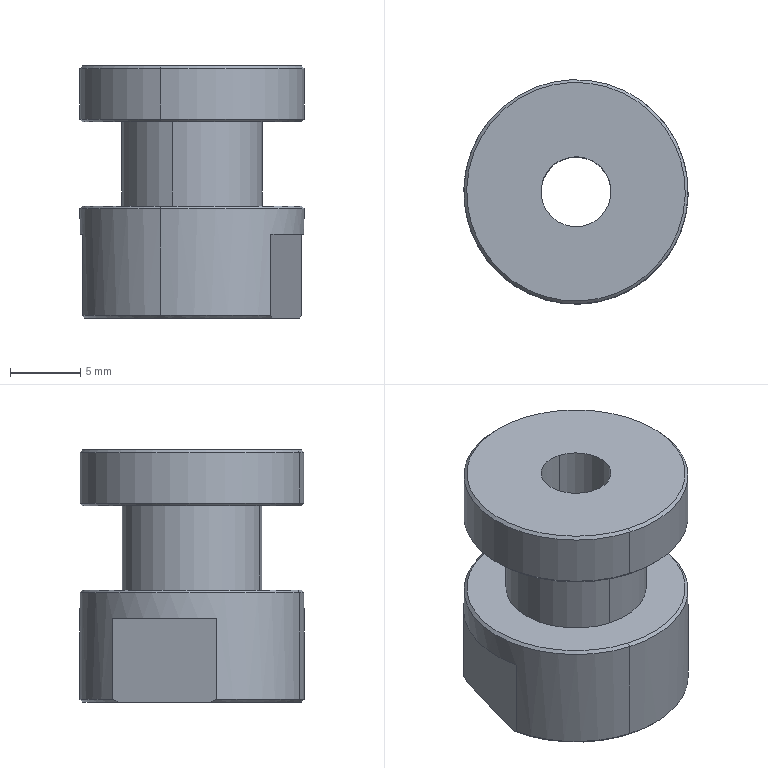Component | SolidWorks | 002MaterialPickingModuleA-1_004SidePlugModule-1_J-012-1 | 1 solid | 25 faces | box 16 x 16 x 18 mm | volume 2464 mm3 | cone 9 | cylinder 8 | plane 8 | commonest cylinder face diameters 16 x4 5 x2 10 x2 | material 45
build123d program:
from build123d import *

# Parameters (mm, degrees)
M6_TAPPED_HOLE1_D  = 5
CUT_EXTRUDE1_DEPTH = 6
CHAMFER1_SIZE      = 0.2


with BuildPart() as part:
    # Sketch2 → Revolve1 (revolve)
    with BuildSketch(Plane.XY, mode=Mode.PRIVATE) as revolve1_sk:
        Polygon((0, 0), (0, 8), (4, 8), (4, 5), (10, 5), (10, 8), (18, 8), (18, 0), align=None)
    revolve(revolve1_sk.sketch.rotate(Axis((0, 0, 0), (1, 0, 0)), 90), axis=Axis((0, 0, 0), (1, 0, 0)))

    # M6 Tapped Hole1 (through all)
    with Locations(Plane(origin=(18, 0, 0), x_dir=(0, 0, -1), z_dir=(1, 0, 0))):
        with Locations((0, 0)):
            Hole(M6_TAPPED_HOLE1_D / 2)

    # Sketch5 → Cut-Extrude1 (cut)
    with BuildSketch(Plane(origin=(18, 0, 0), x_dir=(0, 0, -1), z_dir=(1, 0, 0))):
        with BuildLine():
            Line((3.873, -7), (-3.873, -7))
            ThreePointArc((-3.873, -7), (0, -8), (3.873, -7))
        make_face()
        with BuildLine():
            Line((3.873, 7), (-3.873, 7))
            ThreePointArc((-3.873, 7), (0, 8), (3.873, 7))
        make_face()
    extrude(amount=-CUT_EXTRUDE1_DEPTH, mode=Mode.SUBTRACT)

    # Chamfer1
    chamfer1_edges = [part.edges().sort_by_distance(p)[0] for p in [
        (18, 0, -8),
        (18, -4.063, 6.891),
        (10, 0, -8),
        (4, 0, -8),
        (0, 0, -8),
    ]]
    chamfer(chamfer1_edges, length=CHAMFER1_SIZE)


solid = part.part

# Placed as in the assembly
solid = solid.moved(Location((220.325, 319.019, 480.731), (-90, 16.272, 90)))
STEP:
#1=COLOUR_RGB('',0.7922,0.8196,0.9333);
#2=FILL_AREA_STYLE_COLOUR('',#1);
#3=FILL_AREA_STYLE('',(#2));
#4=SURFACE_STYLE_FILL_AREA(#3);
#5=SURFACE_SIDE_STYLE('',(#4));
#6=SURFACE_STYLE_USAGE(.BOTH.,#5);
#7=PRESENTATION_STYLE_ASSIGNMENT((#6));
#8=CARTESIAN_POINT('',(8.76,12.855,18.218));
#9=VERTEX_POINT('',#8);
#10=CARTESIAN_POINT('',(8.977,12.613,18.218));
#11=VERTEX_POINT('',#10);
#12=CARTESIAN_POINT('',(8.674,12.56,18.218));
#13=DIRECTION('',(0.,0.,-1.));
#14=DIRECTION('',(0.2802,0.9599,0.));
#15=AXIS2_PLACEMENT_3D('',#12,#13,#14);
#16=CIRCLE('',#15,0.3071);
#17=EDGE_CURVE('',#9,#11,#16,.T.);
#18=ORIENTED_EDGE('',*,*,#17,.F.);
#19=CARTESIAN_POINT('',(8.762,12.862,18.226));
#20=VERTEX_POINT('',#19);
#21=CARTESIAN_POINT('',(8.762,12.862,18.226));
#22=DIRECTION('',(0.1981,0.6788,0.7071));
#23=VECTOR('',#22,39.37);
#24=LINE('',#21,#23);
#25=EDGE_CURVE('',#9,#20,#24,.T.);
#26=ORIENTED_EDGE('',*,*,#25,.T.);
#27=CARTESIAN_POINT('',(8.981,12.629,18.226));
#28=VERTEX_POINT('',#27);
#29=CARTESIAN_POINT('',(8.674,12.56,18.226));
#30=DIRECTION('',(0.,0.,1.));
#31=DIRECTION('',(0.2802,0.9599,0.));
#32=AXIS2_PLACEMENT_3D('',#29,#30,#31);
#33=CIRCLE('',#32,0.315);
#34=EDGE_CURVE('',#28,#20,#33,.T.);
#35=ORIENTED_EDGE('',*,*,#34,.F.);
#36=CARTESIAN_POINT('',(8.977,12.613,18.218));
#37=CARTESIAN_POINT('',(8.978,12.618,18.22));
#38=CARTESIAN_POINT('',(8.98,12.624,18.223));
#39=CARTESIAN_POINT('',(8.981,12.629,18.226));
#40=B_SPLINE_CURVE_WITH_KNOTS('',3,(#36,#37,#38,#39),.UNSPECIFIED.,.F.,.F.,(4,4),(0.,0.0004761),.UNSPECIFIED.);
#41=EDGE_CURVE('',#11,#28,#40,.T.);
#42=ORIENTED_EDGE('',*,*,#41,.F.);
#43=EDGE_LOOP('',(#18,#26,#35,#42));
#44=FACE_OUTER_BOUND('',#43,.T.);
#45=CARTESIAN_POINT('',(8.674,12.56,18.226));
#46=DIRECTION('',(0.,0.,1.));
#47=DIRECTION('',(0.2802,0.9599,0.));
#48=AXIS2_PLACEMENT_3D('',#45,#46,#47);
#49=CONICAL_SURFACE('',#48,0.315,0.7854);
#50=ADVANCED_FACE('',(#44),#49,.T.);
#51=CARTESIAN_POINT('',(8.76,12.855,18.533));
#52=VERTEX_POINT('',#51);
#53=CARTESIAN_POINT('',(8.588,12.265,18.533));
#54=VERTEX_POINT('',#53);
#55=CARTESIAN_POINT('',(8.674,12.56,18.533));
#56=DIRECTION('',(0.,0.,1.));
#57=DIRECTION('',(-0.2802,-0.9599,0.));
#58=AXIS2_PLACEMENT_3D('',#55,#56,#57);
#59=CIRCLE('',#58,0.3071);
#60=EDGE_CURVE('',#52,#54,#59,.T.);
#61=ORIENTED_EDGE('',*,*,#60,.F.);
#62=CARTESIAN_POINT('',(8.762,12.862,18.525));
#63=VERTEX_POINT('',#62);
#64=CARTESIAN_POINT('',(8.76,12.855,18.533));
#65=DIRECTION('',(0.1981,0.6788,-0.7071));
#66=VECTOR('',#65,39.37);
#67=LINE('',#64,#66);
#68=EDGE_CURVE('',#52,#63,#67,.T.);
#69=ORIENTED_EDGE('',*,*,#68,.T.);
#70=CARTESIAN_POINT('',(8.586,12.257,18.525));
#71=VERTEX_POINT('',#70);
#72=CARTESIAN_POINT('',(8.674,12.56,18.525));
#73=DIRECTION('',(0.,0.,-1.));
#74=DIRECTION('',(-0.2802,-0.9599,0.));
#75=AXIS2_PLACEMENT_3D('',#72,#73,#74);
#76=CIRCLE('',#75,0.315);
#77=EDGE_CURVE('',#71,#63,#76,.T.);
#78=ORIENTED_EDGE('',*,*,#77,.F.);
#79=CARTESIAN_POINT('',(8.588,12.265,18.533));
#80=DIRECTION('',(-0.1981,-0.6788,-0.7071));
#81=VECTOR('',#80,39.37);
#82=LINE('',#79,#81);
#83=EDGE_CURVE('',#54,#71,#82,.T.);
#84=ORIENTED_EDGE('',*,*,#83,.F.);
#85=EDGE_LOOP('',(#61,#69,#78,#84));
#86=FACE_OUTER_BOUND('',#85,.T.);
#87=CARTESIAN_POINT('',(8.674,12.56,18.533));
#88=DIRECTION('',(0.,0.,-1.));
#89=DIRECTION('',(-0.2802,-0.9599,0.));
#90=AXIS2_PLACEMENT_3D('',#87,#88,#89);
#91=CONICAL_SURFACE('',#90,0.3071,0.7854);
#92=ADVANCED_FACE('',(#86),#91,.T.);
#93=CARTESIAN_POINT('',(8.588,12.265,18.769));
#94=VERTEX_POINT('',#93);
#95=CARTESIAN_POINT('',(8.76,12.855,18.769));
#96=VERTEX_POINT('',#95);
#97=CARTESIAN_POINT('',(8.674,12.56,18.769));
#98=DIRECTION('',(0.,0.,-1.));
#99=DIRECTION('',(0.2802,0.9599,0.));
#100=AXIS2_PLACEMENT_3D('',#97,#98,#99);
#101=CIRCLE('',#100,0.3071);
#102=EDGE_CURVE('',#94,#96,#101,.T.);
#103=ORIENTED_EDGE('',*,*,#102,.F.);
#104=CARTESIAN_POINT('',(8.586,12.257,18.777));
#105=VERTEX_POINT('',#104);
#106=CARTESIAN_POINT('',(8.586,12.257,18.777));
#107=DIRECTION('',(-0.1981,-0.6788,0.7071));
#108=VECTOR('',#107,39.37);
#109=LINE('',#106,#108);
#110=EDGE_CURVE('',#94,#105,#109,.T.);
#111=ORIENTED_EDGE('',*,*,#110,.T.);
#112=CARTESIAN_POINT('',(8.762,12.862,18.777));
#113=VERTEX_POINT('',#112);
#114=CARTESIAN_POINT('',(8.674,12.56,18.777));
#115=DIRECTION('',(0.,0.,1.));
#116=DIRECTION('',(0.2802,0.9599,0.));
#117=AXIS2_PLACEMENT_3D('',#114,#115,#116);
#118=CIRCLE('',#117,0.315);
#119=EDGE_CURVE('',#113,#105,#118,.T.);
#120=ORIENTED_EDGE('',*,*,#119,.F.);
#121=CARTESIAN_POINT('',(8.762,12.862,18.777));
#122=DIRECTION('',(0.1981,0.6788,0.7071));
#123=VECTOR('',#122,39.37);
#124=LINE('',#121,#123);
#125=EDGE_CURVE('',#96,#113,#124,.T.);
#126=ORIENTED_EDGE('',*,*,#125,.F.);
#127=EDGE_LOOP('',(#103,#111,#120,#126));
#128=FACE_OUTER_BOUND('',#127,.T.);
#129=CARTESIAN_POINT('',(8.674,12.56,18.777));
#130=DIRECTION('',(0.,0.,1.));
#131=DIRECTION('',(0.2802,0.9599,0.));
#132=AXIS2_PLACEMENT_3D('',#129,#130,#131);
#133=CONICAL_SURFACE('',#132,0.315,0.7854);
#134=ADVANCED_FACE('',(#128),#133,.T.);
#135=CARTESIAN_POINT('',(8.76,12.855,18.926));
#136=VERTEX_POINT('',#135);
#137=CARTESIAN_POINT('',(8.588,12.265,18.926));
#138=VERTEX_POINT('',#137);
#139=CARTESIAN_POINT('',(8.674,12.56,18.926));
#140=DIRECTION('',(0.,0.,1.));
#141=DIRECTION('',(-0.2802,-0.9599,0.));
#142=AXIS2_PLACEMENT_3D('',#139,#140,#141);
#143=CIRCLE('',#142,0.3071);
#144=EDGE_CURVE('',#136,#138,#143,.T.);
#145=ORIENTED_EDGE('',*,*,#144,.F.);
#146=CARTESIAN_POINT('',(8.762,12.862,18.919));
#147=VERTEX_POINT('',#146);
#148=CARTESIAN_POINT('',(8.76,12.855,18.926));
#149=DIRECTION('',(0.1981,0.6788,-0.7071));
#150=VECTOR('',#149,39.37);
#151=LINE('',#148,#150);
#152=EDGE_CURVE('',#136,#147,#151,.T.);
#153=ORIENTED_EDGE('',*,*,#152,.T.);
#154=CARTESIAN_POINT('',(8.586,12.257,18.919));
#155=VERTEX_POINT('',#154);
#156=CARTESIAN_POINT('',(8.674,12.56,18.919));
#157=DIRECTION('',(0.,0.,-1.));
#158=DIRECTION('',(-0.2802,-0.9599,0.));
#159=AXIS2_PLACEMENT_3D('',#156,#157,#158);
#160=CIRCLE('',#159,0.315);
#161=EDGE_CURVE('',#155,#147,#160,.T.);
#162=ORIENTED_EDGE('',*,*,#161,.F.);
#163=CARTESIAN_POINT('',(8.588,12.265,18.926));
#164=DIRECTION('',(-0.1981,-0.6788,-0.7071));
#165=VECTOR('',#164,39.37);
#166=LINE('',#163,#165);
#167=EDGE_CURVE('',#138,#155,#166,.T.);
#168=ORIENTED_EDGE('',*,*,#167,.F.);
#169=EDGE_LOOP('',(#145,#153,#162,#168));
#170=FACE_OUTER_BOUND('',#169,.T.);
#171=CARTESIAN_POINT('',(8.674,12.56,18.926));
#172=DIRECTION('',(0.,0.,-1.));
#173=DIRECTION('',(-0.2802,-0.9599,0.));
#174=AXIS2_PLACEMENT_3D('',#171,#172,#173);
#175=CONICAL_SURFACE('',#174,0.3071,0.7854);
#176=ADVANCED_FACE('',(#170),#175,.T.);
#177=CARTESIAN_POINT('',(8.702,12.654,18.926));
#178=VERTEX_POINT('',#177);
#179=CARTESIAN_POINT('',(8.647,12.465,18.926));
#180=VERTEX_POINT('',#179);
#181=CARTESIAN_POINT('',(8.674,12.56,18.926));
#182=DIRECTION('',(0.,0.,-1.));
#183=DIRECTION('',(-0.2802,-0.9599,0.));
#184=AXIS2_PLACEMENT_3D('',#181,#182,#183);
#185=CIRCLE('',#184,0.09843);
#186=EDGE_CURVE('',#178,#180,#185,.T.);
#187=ORIENTED_EDGE('',*,*,#186,.F.);
#188=CARTESIAN_POINT('',(8.702,12.654,18.218));
#189=VERTEX_POINT('',#188);
#190=CARTESIAN_POINT('',(8.702,12.654,18.218));
#191=DIRECTION('',(0.,0.,-1.));
#192=VECTOR('',#191,39.37);
#193=LINE('',#190,#192);
#194=EDGE_CURVE('',#178,#189,#193,.T.);
#195=ORIENTED_EDGE('',*,*,#194,.T.);
#196=CARTESIAN_POINT('',(8.647,12.465,18.218));
#197=VERTEX_POINT('',#196);
#198=CARTESIAN_POINT('',(8.674,12.56,18.218));
#199=DIRECTION('',(0.,0.,-1.));
#200=DIRECTION('',(-0.2802,-0.9599,0.));
#201=AXIS2_PLACEMENT_3D('',#198,#199,#200);
#202=CIRCLE('',#201,0.09843);
#203=EDGE_CURVE('',#189,#197,#202,.T.);
#204=ORIENTED_EDGE('',*,*,#203,.T.);
#205=CARTESIAN_POINT('',(8.647,12.465,18.218));
#206=DIRECTION('',(0.,0.,-1.));
#207=VECTOR('',#206,39.37);
#208=LINE('',#205,#207);
#209=EDGE_CURVE('',#180,#197,#208,.T.);
#210=ORIENTED_EDGE('',*,*,#209,.F.);
#211=EDGE_LOOP('',(#187,#195,#204,#210));
#212=FACE_OUTER_BOUND('',#211,.T.);
#213=CARTESIAN_POINT('',(8.674,12.56,18.218));
#214=DIRECTION('',(0.,0.,-1.));
#215=DIRECTION('',(-0.2802,-0.9599,0.));
#216=AXIS2_PLACEMENT_3D('',#213,#214,#215);
#217=CYLINDRICAL_SURFACE('',#216,0.09843);
#218=ADVANCED_FACE('',(#212),#217,.F.);
#219=CARTESIAN_POINT('',(8.367,12.491,18.226));
#220=VERTEX_POINT('',#219);
#221=CARTESIAN_POINT('',(8.586,12.257,18.226));
#222=VERTEX_POINT('',#221);
#223=CARTESIAN_POINT('',(8.674,12.56,18.226));
#224=DIRECTION('',(0.,0.,1.));
#225=DIRECTION('',(0.2802,0.9599,0.));
#226=AXIS2_PLACEMENT_3D('',#223,#224,#225);
#227=CIRCLE('',#226,0.315);
#228=EDGE_CURVE('',#220,#222,#227,.T.);
#229=ORIENTED_EDGE('',*,*,#228,.T.);
#230=CARTESIAN_POINT('',(8.586,12.257,18.926));
#231=DIRECTION('',(0.,0.,1.));
#232=VECTOR('',#231,39.37);
#233=LINE('',#230,#232);
#234=EDGE_CURVE('',#222,#71,#233,.T.);
#235=ORIENTED_EDGE('',*,*,#234,.T.);
#236=ORIENTED_EDGE('',*,*,#77,.T.);
#237=CARTESIAN_POINT('',(8.762,12.862,18.926));
#238=DIRECTION('',(0.,0.,1.));
#239=VECTOR('',#238,39.37);
#240=LINE('',#237,#239);
#241=EDGE_CURVE('',#20,#63,#240,.T.);
#242=ORIENTED_EDGE('',*,*,#241,.F.);
#243=CARTESIAN_POINT('',(8.452,12.783,18.226));
#244=VERTEX_POINT('',#243);
#245=CARTESIAN_POINT('',(8.674,12.56,18.226));
#246=DIRECTION('',(0.,0.,1.));
#247=DIRECTION('',(0.2802,0.9599,0.));
#248=AXIS2_PLACEMENT_3D('',#245,#246,#247);
#249=CIRCLE('',#248,0.315);
#250=EDGE_CURVE('',#20,#244,#249,.T.);
#251=ORIENTED_EDGE('',*,*,#250,.T.);
#252=CARTESIAN_POINT('',(8.452,12.783,18.454));
#253=VERTEX_POINT('',#252);
#254=CARTESIAN_POINT('',(8.452,12.783,18.454));
#255=DIRECTION('',(0.,0.,-1.));
#256=VECTOR('',#255,39.37);
#257=LINE('',#254,#256);
#258=EDGE_CURVE('',#253,#244,#257,.T.);
#259=ORIENTED_EDGE('',*,*,#258,.F.);
#260=CARTESIAN_POINT('',(8.367,12.491,18.454));
#261=VERTEX_POINT('',#260);
#262=CARTESIAN_POINT('',(8.674,12.56,18.454));
#263=DIRECTION('',(0.,0.,-1.));
#264=DIRECTION('',(-0.2802,-0.9599,0.));
#265=AXIS2_PLACEMENT_3D('',#262,#263,#264);
#266=CIRCLE('',#265,0.315);
#267=EDGE_CURVE('',#261,#253,#266,.T.);
#268=ORIENTED_EDGE('',*,*,#267,.F.);
#269=CARTESIAN_POINT('',(8.367,12.491,18.454));
#270=DIRECTION('',(0.,0.,-1.));
#271=VECTOR('',#270,39.37);
#272=LINE('',#269,#271);
#273=EDGE_CURVE('',#261,#220,#272,.T.);
#274=ORIENTED_EDGE('',*,*,#273,.T.);
#275=EDGE_LOOP('',(#229,#235,#236,#242,#251,#259,#268,#274));
#276=FACE_OUTER_BOUND('',#275,.T.);
#277=CARTESIAN_POINT('',(8.674,12.56,18.926));
#278=DIRECTION('',(0.,0.,1.));
#279=DIRECTION('',(0.2802,0.9599,0.));
#280=AXIS2_PLACEMENT_3D('',#277,#278,#279);
#281=CYLINDRICAL_SURFACE('',#280,0.315);
#282=ADVANCED_FACE('',(#276),#281,.T.);
#283=CARTESIAN_POINT('',(8.729,12.749,18.533));
#284=VERTEX_POINT('',#283);
#285=CARTESIAN_POINT('',(8.619,12.371,18.533));
#286=VERTEX_POINT('',#285);
#287=CARTESIAN_POINT('',(8.674,12.56,18.533));
#288=DIRECTION('',(0.,0.,1.));
#289=DIRECTION('',(0.2802,0.9599,0.));
#290=AXIS2_PLACEMENT_3D('',#287,#288,#289);
#291=CIRCLE('',#290,0.1969);
#292=EDGE_CURVE('',#284,#286,#291,.T.);
#293=ORIENTED_EDGE('',*,*,#292,.T.);
#294=CARTESIAN_POINT('',(8.619,12.371,18.769));
#295=VERTEX_POINT('',#294);
#296=CARTESIAN_POINT('',(8.619,12.371,18.926));
#297=DIRECTION('',(0.,0.,1.));
#298=VECTOR('',#297,39.37);
#299=LINE('',#296,#298);
#300=EDGE_CURVE('',#286,#295,#299,.T.);
#301=ORIENTED_EDGE('',*,*,#300,.T.);
#302=CARTESIAN_POINT('',(8.729,12.749,18.769));
#303=VERTEX_POINT('',#302);
#304=CARTESIAN_POINT('',(8.674,12.56,18.769));
#305=DIRECTION('',(0.,0.,1.));
#306=DIRECTION('',(0.2802,0.9599,0.));
#307=AXIS2_PLACEMENT_3D('',#304,#305,#306);
#308=CIRCLE('',#307,0.1969);
#309=EDGE_CURVE('',#303,#295,#308,.T.);
#310=ORIENTED_EDGE('',*,*,#309,.F.);
#311=CARTESIAN_POINT('',(8.729,12.749,18.926));
#312=DIRECTION('',(0.,0.,1.));
#313=VECTOR('',#312,39.37);
#314=LINE('',#311,#313);
#315=EDGE_CURVE('',#284,#303,#314,.T.);
#316=ORIENTED_EDGE('',*,*,#315,.F.);
#317=EDGE_LOOP('',(#293,#301,#310,#316));
#318=FACE_OUTER_BOUND('',#317,.T.);
#319=CARTESIAN_POINT('',(8.674,12.56,18.926));
#320=DIRECTION('',(0.,0.,1.));
#321=DIRECTION('',(0.2802,0.9599,0.));
#322=AXIS2_PLACEMENT_3D('',#319,#320,#321);
#323=CYLINDRICAL_SURFACE('',#322,0.1969);
#324=ADVANCED_FACE('',(#318),#323,.T.);
#325=ORIENTED_EDGE('',*,*,#119,.T.);
#326=CARTESIAN_POINT('',(8.586,12.257,18.926));
#327=DIRECTION('',(0.,0.,1.));
#328=VECTOR('',#327,39.37);
#329=LINE('',#326,#328);
#330=EDGE_CURVE('',#105,#155,#329,.T.);
#331=ORIENTED_EDGE('',*,*,#330,.T.);
#332=ORIENTED_EDGE('',*,*,#161,.T.);
#333=CARTESIAN_POINT('',(8.762,12.862,18.926));
#334=DIRECTION('',(0.,0.,1.));
#335=VECTOR('',#334,39.37);
#336=LINE('',#333,#335);
#337=EDGE_CURVE('',#113,#147,#336,.T.);
#338=ORIENTED_EDGE('',*,*,#337,.F.);
#339=EDGE_LOOP('',(#325,#331,#332,#338));
#340=FACE_OUTER_BOUND('',#339,.T.);
#341=CARTESIAN_POINT('',(8.674,12.56,18.926));
#342=DIRECTION('',(0.,0.,1.));
#343=DIRECTION('',(0.2802,0.9599,0.));
#344=AXIS2_PLACEMENT_3D('',#341,#342,#343);
#345=CYLINDRICAL_SURFACE('',#344,0.315);
#346=ADVANCED_FACE('',(#340),#345,.T.);
#347=CARTESIAN_POINT('',(8.674,12.56,18.926));
#348=DIRECTION('',(0.,0.,1.));
#349=DIRECTION('',(-0.2802,-0.9599,0.));
#350=AXIS2_PLACEMENT_3D('',#347,#348,#349);
#351=CIRCLE('',#350,0.3071);
#352=EDGE_CURVE('',#138,#136,#351,.T.);
#353=ORIENTED_EDGE('',*,*,#352,.T.);
#354=ORIENTED_EDGE('',*,*,#144,.T.);
#355=EDGE_LOOP('',(#353,#354));
#356=FACE_OUTER_BOUND('',#355,.T.);
#357=CARTESIAN_POINT('',(8.674,12.56,18.926));
#358=DIRECTION('',(0.,0.,-1.));
#359=DIRECTION('',(-0.2802,-0.9599,0.));
#360=AXIS2_PLACEMENT_3D('',#357,#358,#359);
#361=CIRCLE('',#360,0.09843);
#362=EDGE_CURVE('',#180,#178,#361,.T.);
#363=ORIENTED_EDGE('',*,*,#362,.T.);
#364=ORIENTED_EDGE('',*,*,#186,.T.);
#365=EDGE_LOOP('',(#363,#364));
#366=FACE_BOUND('',#365,.T.);
#367=CARTESIAN_POINT('',(8.674,12.56,18.926));
#368=DIRECTION('',(0.,0.,-1.));
#369=DIRECTION('',(-0.2802,-0.9599,0.));
#370=AXIS2_PLACEMENT_3D('',#367,#368,#369);
#371=PLANE('',#370);
#372=ADVANCED_FACE('',(#356,#366),#371,.F.);
#373=ORIENTED_EDGE('',*,*,#330,.F.);
#374=CARTESIAN_POINT('',(8.674,12.56,18.777));
#375=DIRECTION('',(0.,0.,1.));
#376=DIRECTION('',(0.2802,0.9599,0.));
#377=AXIS2_PLACEMENT_3D('',#374,#375,#376);
#378=CIRCLE('',#377,0.315);
#379=EDGE_CURVE('',#105,#113,#378,.T.);
#380=ORIENTED_EDGE('',*,*,#379,.T.);
#381=ORIENTED_EDGE('',*,*,#337,.T.);
#382=CARTESIAN_POINT('',(8.674,12.56,18.919));
#383=DIRECTION('',(0.,0.,-1.));
#384=DIRECTION('',(-0.2802,-0.9599,0.));
#385=AXIS2_PLACEMENT_3D('',#382,#383,#384);
#386=CIRCLE('',#385,0.315);
#387=EDGE_CURVE('',#147,#155,#386,.T.);
#388=ORIENTED_EDGE('',*,*,#387,.T.);
#389=EDGE_LOOP('',(#373,#380,#381,#388));
#390=FACE_OUTER_BOUND('',#389,.T.);
#391=CARTESIAN_POINT('',(8.674,12.56,18.926));
#392=DIRECTION('',(0.,0.,1.));
#393=DIRECTION('',(0.2802,0.9599,0.));
#394=AXIS2_PLACEMENT_3D('',#391,#392,#393);
#395=CYLINDRICAL_SURFACE('',#394,0.315);
#396=ADVANCED_FACE('',(#390),#395,.T.);
#397=CARTESIAN_POINT('',(8.674,12.56,18.769));
#398=DIRECTION('',(0.,0.,-1.));
#399=DIRECTION('',(0.2802,0.9599,0.));
#400=AXIS2_PLACEMENT_3D('',#397,#398,#399);
#401=CIRCLE('',#400,0.3071);
#402=EDGE_CURVE('',#96,#94,#401,.T.);
#403=ORIENTED_EDGE('',*,*,#402,.T.);
#404=ORIENTED_EDGE('',*,*,#102,.T.);
#405=EDGE_LOOP('',(#403,#404));
#406=FACE_OUTER_BOUND('',#405,.T.);
#407=ORIENTED_EDGE('',*,*,#309,.T.);
#408=CARTESIAN_POINT('',(8.674,12.56,18.769));
#409=DIRECTION('',(0.,0.,1.));
#410=DIRECTION('',(0.2802,0.9599,0.));
#411=AXIS2_PLACEMENT_3D('',#408,#409,#410);
#412=CIRCLE('',#411,0.1969);
#413=EDGE_CURVE('',#295,#303,#412,.T.);
#414=ORIENTED_EDGE('',*,*,#413,.T.);
#415=EDGE_LOOP('',(#407,#414));
#416=FACE_BOUND('',#415,.T.);
#417=CARTESIAN_POINT('',(8.372,12.648,18.769));
#418=DIRECTION('',(0.,0.,1.));
#419=DIRECTION('',(0.2802,0.9599,0.));
#420=AXIS2_PLACEMENT_3D('',#417,#418,#419);
#421=PLANE('',#420);
#422=ADVANCED_FACE('',(#406,#416),#421,.F.);
#423=ORIENTED_EDGE('',*,*,#300,.F.);
#424=CARTESIAN_POINT('',(8.674,12.56,18.533));
#425=DIRECTION('',(0.,0.,1.));
#426=DIRECTION('',(0.2802,0.9599,0.));
#427=AXIS2_PLACEMENT_3D('',#424,#425,#426);
#428=CIRCLE('',#427,0.1969);
#429=EDGE_CURVE('',#286,#284,#428,.T.);
#430=ORIENTED_EDGE('',*,*,#429,.T.);
#431=ORIENTED_EDGE('',*,*,#315,.T.);
#432=ORIENTED_EDGE('',*,*,#413,.F.);
#433=EDGE_LOOP('',(#423,#430,#431,#432));
#434=FACE_OUTER_BOUND('',#433,.T.);
#435=CARTESIAN_POINT('',(8.674,12.56,18.926));
#436=DIRECTION('',(0.,0.,1.));
#437=DIRECTION('',(0.2802,0.9599,0.));
#438=AXIS2_PLACEMENT_3D('',#435,#436,#437);
#439=CYLINDRICAL_SURFACE('',#438,0.1969);
#440=ADVANCED_FACE('',(#434),#439,.T.);
#441=CARTESIAN_POINT('',(8.674,12.56,18.533));
#442=DIRECTION('',(0.,0.,1.));
#443=DIRECTION('',(-0.2802,-0.9599,0.));
#444=AXIS2_PLACEMENT_3D('',#441,#442,#443);
#445=CIRCLE('',#444,0.3071);
#446=EDGE_CURVE('',#54,#52,#445,.T.);
#447=ORIENTED_EDGE('',*,*,#446,.T.);
#448=ORIENTED_EDGE('',*,*,#60,.T.);
#449=EDGE_LOOP('',(#447,#448));
#450=FACE_OUTER_BOUND('',#449,.T.);
#451=ORIENTED_EDGE('',*,*,#292,.F.);
#452=ORIENTED_EDGE('',*,*,#429,.F.);
#453=EDGE_LOOP('',(#451,#452));
#454=FACE_BOUND('',#453,.T.);
#455=CARTESIAN_POINT('',(8.485,12.615,18.533));
#456=DIRECTION('',(0.,0.,-1.));
#457=DIRECTION('',(-0.2802,-0.9599,0.));
#458=AXIS2_PLACEMENT_3D('',#455,#456,#457);
#459=PLANE('',#458);
#460=ADVANCED_FACE('',(#450,#454),#459,.F.);
#461=ORIENTED_EDGE('',*,*,#234,.F.);
#462=CARTESIAN_POINT('',(8.896,12.336,18.226));
#463=VERTEX_POINT('',#462);
#464=CARTESIAN_POINT('',(8.674,12.56,18.226));
#465=DIRECTION('',(0.,0.,1.));
#466=DIRECTION('',(0.2802,0.9599,0.));
#467=AXIS2_PLACEMENT_3D('',#464,#465,#466);
#468=CIRCLE('',#467,0.315);
#469=EDGE_CURVE('',#222,#463,#468,.T.);
#470=ORIENTED_EDGE('',*,*,#469,.T.);
#471=CARTESIAN_POINT('',(8.896,12.336,18.454));
#472=VERTEX_POINT('',#471);
#473=CARTESIAN_POINT('',(8.896,12.336,18.454));
#474=DIRECTION('',(0.,0.,-1.));
#475=VECTOR('',#474,39.37);
#476=LINE('',#473,#475);
#477=EDGE_CURVE('',#472,#463,#476,.T.);
#478=ORIENTED_EDGE('',*,*,#477,.F.);
#479=CARTESIAN_POINT('',(8.981,12.629,18.454));
#480=VERTEX_POINT('',#479);
#481=CARTESIAN_POINT('',(8.674,12.56,18.454));
#482=DIRECTION('',(0.,0.,-1.));
#483=DIRECTION('',(-0.2802,-0.9599,0.));
#484=AXIS2_PLACEMENT_3D('',#481,#482,#483);
#485=CIRCLE('',#484,0.315);
#486=EDGE_CURVE('',#480,#472,#485,.T.);
#487=ORIENTED_EDGE('',*,*,#486,.F.);
#488=CARTESIAN_POINT('',(8.981,12.629,18.454));
#489=DIRECTION('',(0.,0.,-1.));
#490=VECTOR('',#489,39.37);
#491=LINE('',#488,#490);
#492=EDGE_CURVE('',#480,#28,#491,.T.);
#493=ORIENTED_EDGE('',*,*,#492,.T.);
#494=ORIENTED_EDGE('',*,*,#34,.T.);
#495=ORIENTED_EDGE('',*,*,#241,.T.);
#496=CARTESIAN_POINT('',(8.674,12.56,18.525));
#497=DIRECTION('',(0.,0.,-1.));
#498=DIRECTION('',(-0.2802,-0.9599,0.));
#499=AXIS2_PLACEMENT_3D('',#496,#497,#498);
#500=CIRCLE('',#499,0.315);
#501=EDGE_CURVE('',#63,#71,#500,.T.);
#502=ORIENTED_EDGE('',*,*,#501,.T.);
#503=EDGE_LOOP('',(#461,#470,#478,#487,#493,#494,#495,#502));
#504=FACE_OUTER_BOUND('',#503,.T.);
#505=CARTESIAN_POINT('',(8.674,12.56,18.926));
#506=DIRECTION('',(0.,0.,1.));
#507=DIRECTION('',(0.2802,0.9599,0.));
#508=AXIS2_PLACEMENT_3D('',#505,#506,#507);
#509=CYLINDRICAL_SURFACE('',#508,0.315);
#510=ADVANCED_FACE('',(#504),#509,.T.);
#511=CARTESIAN_POINT('',(8.674,12.56,18.218));
#512=DIRECTION('',(0.,0.,-1.));
#513=DIRECTION('',(-0.2802,-0.9599,0.));
#514=AXIS2_PLACEMENT_3D('',#511,#512,#513);
#515=CIRCLE('',#514,0.09843);
#516=EDGE_CURVE('',#197,#189,#515,.T.);
#517=ORIENTED_EDGE('',*,*,#516,.F.);
#518=ORIENTED_EDGE('',*,*,#203,.F.);
#519=EDGE_LOOP('',(#517,#518));
#520=FACE_BOUND('',#519,.T.);
#521=CARTESIAN_POINT('',(8.448,12.767,18.218));
#522=VERTEX_POINT('',#521);
#523=CARTESIAN_POINT('',(8.372,12.507,18.218));
#524=VERTEX_POINT('',#523);
#525=CARTESIAN_POINT('',(8.367,12.491,18.218));
#526=DIRECTION('',(-0.2802,-0.9599,0.));
#527=VECTOR('',#526,39.37);
#528=LINE('',#525,#527);
#529=EDGE_CURVE('',#522,#524,#528,.T.);
#530=ORIENTED_EDGE('',*,*,#529,.F.);
#531=CARTESIAN_POINT('',(8.674,12.56,18.218));
#532=DIRECTION('',(0.,0.,-1.));
#533=DIRECTION('',(0.2802,0.9599,0.));
#534=AXIS2_PLACEMENT_3D('',#531,#532,#533);
#535=CIRCLE('',#534,0.3071);
#536=EDGE_CURVE('',#522,#9,#535,.T.);
#537=ORIENTED_EDGE('',*,*,#536,.T.);
#538=ORIENTED_EDGE('',*,*,#17,.T.);
#539=CARTESIAN_POINT('',(8.901,12.353,18.218));
#540=VERTEX_POINT('',#539);
#541=CARTESIAN_POINT('',(8.896,12.336,18.218));
#542=DIRECTION('',(0.2802,0.9599,0.));
#543=VECTOR('',#542,39.37);
#544=LINE('',#541,#543);
#545=EDGE_CURVE('',#540,#11,#544,.T.);
#546=ORIENTED_EDGE('',*,*,#545,.F.);
#547=CARTESIAN_POINT('',(8.674,12.56,18.218));
#548=DIRECTION('',(0.,0.,-1.));
#549=DIRECTION('',(0.2802,0.9599,0.));
#550=AXIS2_PLACEMENT_3D('',#547,#548,#549);
#551=CIRCLE('',#550,0.3071);
#552=EDGE_CURVE('',#540,#524,#551,.T.);
#553=ORIENTED_EDGE('',*,*,#552,.T.);
#554=EDGE_LOOP('',(#530,#537,#538,#546,#553));
#555=FACE_OUTER_BOUND('',#554,.T.);
#556=CARTESIAN_POINT('',(8.372,12.648,18.218));
#557=DIRECTION('',(0.,0.,1.));
#558=DIRECTION('',(0.2802,0.9599,0.));
#559=AXIS2_PLACEMENT_3D('',#556,#557,#558);
#560=PLANE('',#559);
#561=ADVANCED_FACE('',(#520,#555),#560,.F.);
#562=ORIENTED_EDGE('',*,*,#194,.F.);
#563=ORIENTED_EDGE('',*,*,#362,.F.);
#564=ORIENTED_EDGE('',*,*,#209,.T.);
#565=ORIENTED_EDGE('',*,*,#516,.T.);
#566=EDGE_LOOP('',(#562,#563,#564,#565));
#567=FACE_OUTER_BOUND('',#566,.T.);
#568=CARTESIAN_POINT('',(8.674,12.56,18.218));
#569=DIRECTION('',(0.,0.,-1.));
#570=DIRECTION('',(-0.2802,-0.9599,0.));
#571=AXIS2_PLACEMENT_3D('',#568,#569,#570);
#572=CYLINDRICAL_SURFACE('',#571,0.09843);
#573=ADVANCED_FACE('',(#567),#572,.F.);
#574=ORIENTED_EDGE('',*,*,#258,.T.);
#575=CARTESIAN_POINT('',(8.452,12.783,18.226));
#576=CARTESIAN_POINT('',(8.451,12.778,18.223));
#577=CARTESIAN_POINT('',(8.449,12.773,18.22));
#578=CARTESIAN_POINT('',(8.448,12.767,18.218));
#579=B_SPLINE_CURVE_WITH_KNOTS('',3,(#575,#576,#577,#578),.UNSPECIFIED.,.F.,.F.,(4,4),(0.,0.0004761),.UNSPECIFIED.);
#580=EDGE_CURVE('',#244,#522,#579,.T.);
#581=ORIENTED_EDGE('',*,*,#580,.T.);
#582=ORIENTED_EDGE('',*,*,#529,.T.);
#583=CARTESIAN_POINT('',(8.372,12.507,18.218));
#584=CARTESIAN_POINT('',(8.37,12.501,18.22));
#585=CARTESIAN_POINT('',(8.369,12.496,18.223));
#586=CARTESIAN_POINT('',(8.367,12.491,18.226));
#587=B_SPLINE_CURVE_WITH_KNOTS('',3,(#583,#584,#585,#586),.UNSPECIFIED.,.F.,.F.,(4,4),(0.,0.0004761),.UNSPECIFIED.);
#588=EDGE_CURVE('',#524,#220,#587,.T.);
#589=ORIENTED_EDGE('',*,*,#588,.T.);
#590=ORIENTED_EDGE('',*,*,#273,.F.);
#591=CARTESIAN_POINT('',(8.367,12.491,18.454));
#592=DIRECTION('',(-0.2802,-0.9599,0.));
#593=VECTOR('',#592,39.37);
#594=LINE('',#591,#593);
#595=EDGE_CURVE('',#253,#261,#594,.T.);
#596=ORIENTED_EDGE('',*,*,#595,.F.);
#597=EDGE_LOOP('',(#574,#581,#582,#589,#590,#596));
#598=FACE_OUTER_BOUND('',#597,.T.);
#599=CARTESIAN_POINT('',(8.367,12.491,18.454));
#600=DIRECTION('',(0.9599,-0.2802,0.));
#601=DIRECTION('',(-0.2802,-0.9599,0.));
#602=AXIS2_PLACEMENT_3D('',#599,#600,#601);
#603=PLANE('',#602);
#604=ADVANCED_FACE('',(#598),#603,.F.);
#605=ORIENTED_EDGE('',*,*,#267,.T.);
#606=ORIENTED_EDGE('',*,*,#595,.T.);
#607=EDGE_LOOP('',(#605,#606));
#608=FACE_OUTER_BOUND('',#607,.T.);
#609=CARTESIAN_POINT('',(8.674,12.56,18.454));
#610=DIRECTION('',(0.,0.,-1.));
#611=DIRECTION('',(-0.2802,-0.9599,0.));
#612=AXIS2_PLACEMENT_3D('',#609,#610,#611);
#613=PLANE('',#612);
#614=ADVANCED_FACE('',(#608),#613,.T.);
#615=ORIENTED_EDGE('',*,*,#545,.T.);
#616=ORIENTED_EDGE('',*,*,#41,.T.);
#617=ORIENTED_EDGE('',*,*,#492,.F.);
#618=CARTESIAN_POINT('',(8.896,12.336,18.454));
#619=DIRECTION('',(0.2802,0.9599,0.));
#620=VECTOR('',#619,39.37);
#621=LINE('',#618,#620);
#622=EDGE_CURVE('',#472,#480,#621,.T.);
#623=ORIENTED_EDGE('',*,*,#622,.F.);
#624=ORIENTED_EDGE('',*,*,#477,.T.);
#625=CARTESIAN_POINT('',(8.896,12.336,18.226));
#626=CARTESIAN_POINT('',(8.898,12.342,18.223));
#627=CARTESIAN_POINT('',(8.899,12.347,18.22));
#628=CARTESIAN_POINT('',(8.901,12.353,18.218));
#629=B_SPLINE_CURVE_WITH_KNOTS('',3,(#625,#626,#627,#628),.UNSPECIFIED.,.F.,.F.,(4,4),(0.,0.0004761),.UNSPECIFIED.);
#630=EDGE_CURVE('',#463,#540,#629,.T.);
#631=ORIENTED_EDGE('',*,*,#630,.T.);
#632=EDGE_LOOP('',(#615,#616,#617,#623,#624,#631));
#633=FACE_OUTER_BOUND('',#632,.T.);
#634=CARTESIAN_POINT('',(8.896,12.336,18.454));
#635=DIRECTION('',(-0.9599,0.2802,0.));
#636=DIRECTION('',(0.2802,0.9599,0.));
#637=AXIS2_PLACEMENT_3D('',#634,#635,#636);
#638=PLANE('',#637);
#639=ADVANCED_FACE('',(#633),#638,.F.);
#640=ORIENTED_EDGE('',*,*,#486,.T.);
#641=ORIENTED_EDGE('',*,*,#622,.T.);
#642=EDGE_LOOP('',(#640,#641));
#643=FACE_OUTER_BOUND('',#642,.T.);
#644=CARTESIAN_POINT('',(8.674,12.56,18.454));
#645=DIRECTION('',(0.,0.,-1.));
#646=DIRECTION('',(-0.2802,-0.9599,0.));
#647=AXIS2_PLACEMENT_3D('',#644,#645,#646);
#648=PLANE('',#647);
#649=ADVANCED_FACE('',(#643),#648,.T.);
#650=ORIENTED_EDGE('',*,*,#152,.F.);
#651=ORIENTED_EDGE('',*,*,#352,.F.);
#652=ORIENTED_EDGE('',*,*,#167,.T.);
#653=ORIENTED_EDGE('',*,*,#387,.F.);
#654=EDGE_LOOP('',(#650,#651,#652,#653));
#655=FACE_OUTER_BOUND('',#654,.T.);
#656=CARTESIAN_POINT('',(8.674,12.56,18.926));
#657=DIRECTION('',(0.,0.,-1.));
#658=DIRECTION('',(-0.2802,-0.9599,0.));
#659=AXIS2_PLACEMENT_3D('',#656,#657,#658);
#660=CONICAL_SURFACE('',#659,0.3071,0.7854);
#661=ADVANCED_FACE('',(#655),#660,.T.);
#662=ORIENTED_EDGE('',*,*,#110,.F.);
#663=ORIENTED_EDGE('',*,*,#402,.F.);
#664=ORIENTED_EDGE('',*,*,#125,.T.);
#665=ORIENTED_EDGE('',*,*,#379,.F.);
#666=EDGE_LOOP('',(#662,#663,#664,#665));
#667=FACE_OUTER_BOUND('',#666,.T.);
#668=CARTESIAN_POINT('',(8.674,12.56,18.777));
#669=DIRECTION('',(0.,0.,1.));
#670=DIRECTION('',(0.2802,0.9599,0.));
#671=AXIS2_PLACEMENT_3D('',#668,#669,#670);
#672=CONICAL_SURFACE('',#671,0.315,0.7854);
#673=ADVANCED_FACE('',(#667),#672,.T.);
#674=ORIENTED_EDGE('',*,*,#68,.F.);
#675=ORIENTED_EDGE('',*,*,#446,.F.);
#676=ORIENTED_EDGE('',*,*,#83,.T.);
#677=ORIENTED_EDGE('',*,*,#501,.F.);
#678=EDGE_LOOP('',(#674,#675,#676,#677));
#679=FACE_OUTER_BOUND('',#678,.T.);
#680=CARTESIAN_POINT('',(8.674,12.56,18.533));
#681=DIRECTION('',(0.,0.,-1.));
#682=DIRECTION('',(-0.2802,-0.9599,0.));
#683=AXIS2_PLACEMENT_3D('',#680,#681,#682);
#684=CONICAL_SURFACE('',#683,0.3071,0.7854);
#685=ADVANCED_FACE('',(#679),#684,.T.);
#686=ORIENTED_EDGE('',*,*,#25,.F.);
#687=ORIENTED_EDGE('',*,*,#536,.F.);
#688=ORIENTED_EDGE('',*,*,#580,.F.);
#689=ORIENTED_EDGE('',*,*,#250,.F.);
#690=EDGE_LOOP('',(#686,#687,#688,#689));
#691=FACE_OUTER_BOUND('',#690,.T.);
#692=CARTESIAN_POINT('',(8.674,12.56,18.226));
#693=DIRECTION('',(0.,0.,1.));
#694=DIRECTION('',(0.2802,0.9599,0.));
#695=AXIS2_PLACEMENT_3D('',#692,#693,#694);
#696=CONICAL_SURFACE('',#695,0.315,0.7854);
#697=ADVANCED_FACE('',(#691),#696,.T.);
#698=ORIENTED_EDGE('',*,*,#588,.F.);
#699=ORIENTED_EDGE('',*,*,#552,.F.);
#700=ORIENTED_EDGE('',*,*,#630,.F.);
#701=ORIENTED_EDGE('',*,*,#469,.F.);
#702=ORIENTED_EDGE('',*,*,#228,.F.);
#703=EDGE_LOOP('',(#698,#699,#700,#701,#702));
#704=FACE_OUTER_BOUND('',#703,.T.);
#705=CARTESIAN_POINT('',(8.674,12.56,18.226));
#706=DIRECTION('',(0.,0.,1.));
#707=DIRECTION('',(0.2802,0.9599,0.));
#708=AXIS2_PLACEMENT_3D('',#705,#706,#707);
#709=CONICAL_SURFACE('',#708,0.315,0.7854);
#710=ADVANCED_FACE('',(#704),#709,.T.);
#711=CLOSED_SHELL('',(#50,#92,#134,#176,#218,#282,#324,#346,#372,#396,#422,#440,#460,#510,#561,#573,#604,#614,#639,#649,#661,#673,#685,#697,#710));
#712=MANIFOLD_SOLID_BREP('',#711);
#713=STYLED_ITEM('',(#7),#712);
#714=(LENGTH_UNIT()NAMED_UNIT(*)SI_UNIT($,.METRE.));
#715=LENGTH_MEASURE_WITH_UNIT(LENGTH_MEASURE(0.0254),#714);
#716=DIMENSIONAL_EXPONENTS(1.,0.,0.,0.,0.,0.,0.);
#717=(CONVERSION_BASED_UNIT('',#715)LENGTH_UNIT()NAMED_UNIT(#716));
#718=UNCERTAINTY_MEASURE_WITH_UNIT(LENGTH_MEASURE(0.00001),#717,'','');
#719=(NAMED_UNIT(*)PLANE_ANGLE_UNIT()SI_UNIT($,.RADIAN.));
#720=(NAMED_UNIT(*)SI_UNIT($,.STERADIAN.)SOLID_ANGLE_UNIT());
#721=(GEOMETRIC_REPRESENTATION_CONTEXT(3)GLOBAL_UNCERTAINTY_ASSIGNED_CONTEXT((#718))GLOBAL_UNIT_ASSIGNED_CONTEXT((#717,#719,#720))REPRESENTATION_CONTEXT('',''));
#722=MECHANICAL_DESIGN_GEOMETRIC_PRESENTATION_REPRESENTATION('',(#713),#721);
#723=PRESENTATION_LAYER_ASSIGNMENT('','',(#713));
#724=CARTESIAN_POINT('',(0.,0.,0.));
#725=DIRECTION('',(0.,0.,1.));
#726=DIRECTION('',(1.,0.,0.));
#727=AXIS2_PLACEMENT_3D('',#724,#725,#726);
#728=(LENGTH_UNIT()NAMED_UNIT(*)SI_UNIT($,.METRE.));
#729=LENGTH_MEASURE_WITH_UNIT(LENGTH_MEASURE(0.0254),#728);
#730=DIMENSIONAL_EXPONENTS(1.,0.,0.,0.,0.,0.,0.);
#731=(CONVERSION_BASED_UNIT('',#729)LENGTH_UNIT()NAMED_UNIT(#730));
#732=UNCERTAINTY_MEASURE_WITH_UNIT(LENGTH_MEASURE(0.00001),#731,'','');
#733=(NAMED_UNIT(*)PLANE_ANGLE_UNIT()SI_UNIT($,.RADIAN.));
#734=(NAMED_UNIT(*)SI_UNIT($,.STERADIAN.)SOLID_ANGLE_UNIT());
#735=(GEOMETRIC_REPRESENTATION_CONTEXT(3)GLOBAL_UNCERTAINTY_ASSIGNED_CONTEXT((#732))GLOBAL_UNIT_ASSIGNED_CONTEXT((#731,#733,#734))REPRESENTATION_CONTEXT('',''));
#736=ADVANCED_BREP_SHAPE_REPRESENTATION('',(#712,#727),#735);